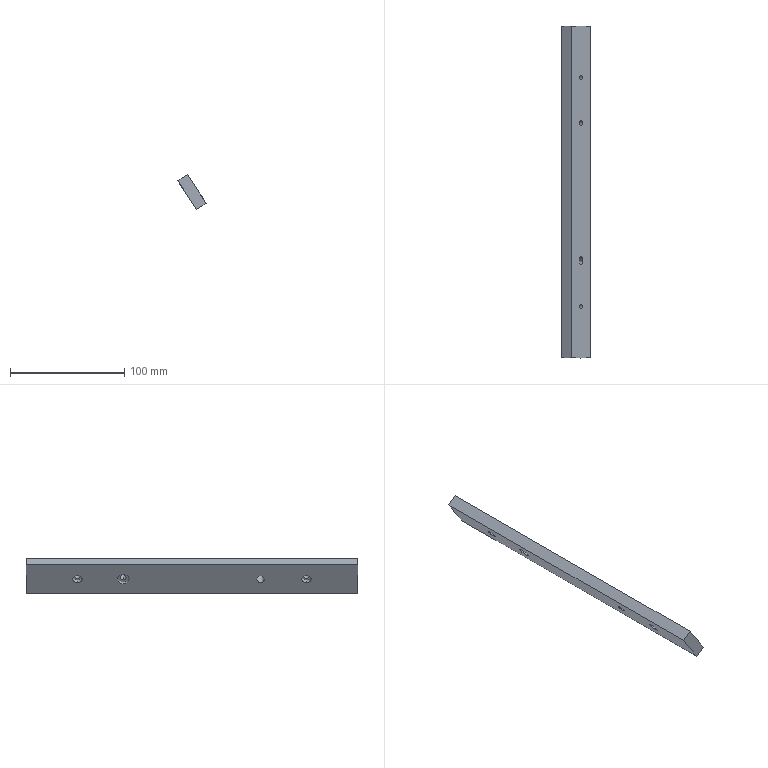Component | SolidWorks | NewSuctionCupGroup-1_SuctionCupMountingPlate-1 | 1 solid | 23 faces | box 24.78 x 290 x 30.58 mm | volume 85630 mm3 | cylinder 14 | plane 9 | commonest cylinder face diameters 8 x4 4.5 x4 5 x2 10 x2 6.8 x2
build123d program:
from build123d import *

# Parameters (mm, degrees)
SKETCH1_W                                            = 290
SKETCH1_H                                            = 30
BOSS_EXTRUDE1_DEPTH                                  = 10
M8_TAPPED_HOLE1_D                                    = 6.8
M8_TAPPED_HOLE1_DEPTH                                = 19.75
M8_TAPPED_HOLE1_TIP                                  = 2.043
SKETCH5_R                                            = 5
CUT_EXTRUDE1_DEPTH                                   = 3
SKETCH6_R                                            = 2.5
CUT_EXTRUDE2_DEPTH                                   = 146.942
HOLE_SIZE_ACCORDING_TO_THE_TYPE_OF_HEXAG_D           = 4.5
HOLE_SIZE_ACCORDING_TO_THE_TYPE_OF_HEXAG_CBORE_D     = 8
HOLE_SIZE_ACCORDING_TO_THE_TYPE_OF_HEXAG_CBORE_DEPTH = 4.6


with BuildPart() as part:
    # Sketch1 → Boss-Extrude1 (new body)
    with BuildSketch(Plane(origin=(0, 0, 0), x_dir=(1, 0, 0), z_dir=(0, 1, 0))):
        Rectangle(SKETCH1_W, SKETCH1_H)
    extrude(amount=BOSS_EXTRUDE1_DEPTH)

    # M8 Tapped Hole1
    with Locations(Plane(origin=(0, 10, 0), x_dir=(1, 0, 0), z_dir=(0, 1, 0))):
        with Locations((60, 0)):
            Hole(M8_TAPPED_HOLE1_D / 2, depth=M8_TAPPED_HOLE1_DEPTH)
            with Locations((0, 0, -(M8_TAPPED_HOLE1_DEPTH + M8_TAPPED_HOLE1_TIP / 2))):  # 118° drill point
                Cone(0, M8_TAPPED_HOLE1_D / 2, M8_TAPPED_HOLE1_TIP, mode=Mode.SUBTRACT)

    # Sketch5 → Cut-Extrude1 (cut)
    with BuildSketch(Plane.XZ):
        with Locations(Location((-60, 0, 0), (0, 0, 270))):
            Circle(SKETCH5_R)
    extrude(amount=-CUT_EXTRUDE1_DEPTH, mode=Mode.SUBTRACT)

    # Sketch6 → Cut-Extrude2 (cut, through all)
    with BuildSketch(Plane.XZ.offset(-3)):
        with Locations(Location((-60, 0, 0), (0, 0, 270))):
            Circle(SKETCH6_R)
    extrude(amount=-CUT_EXTRUDE2_DEPTH, mode=Mode.SUBTRACT)

    # Hole Size according to the type of hexag (through all)
    with Locations(Plane(origin=(0, 0, 0), x_dir=(-1, 0, 0), z_dir=(0, -1, 0))):
        with Locations((100, 0), (-100, 0)):
            CounterBoreHole(HOLE_SIZE_ACCORDING_TO_THE_TYPE_OF_HEXAG_D / 2, HOLE_SIZE_ACCORDING_TO_THE_TYPE_OF_HEXAG_CBORE_D / 2, HOLE_SIZE_ACCORDING_TO_THE_TYPE_OF_HEXAG_CBORE_DEPTH)


solid = part.part

# Placed as in the assembly
solid = solid.moved(Location((-81.422, -40.454, -24.035), (0, -33.165, -90)))
STEP:
#1=COLOUR_RGB('',0.7922,0.8196,0.9333);
#2=FILL_AREA_STYLE_COLOUR('',#1);
#3=FILL_AREA_STYLE('',(#2));
#4=SURFACE_STYLE_FILL_AREA(#3);
#5=SURFACE_SIDE_STYLE('',(#4));
#6=SURFACE_STYLE_USAGE(.BOTH.,#5);
#7=PRESENTATION_STYLE_ASSIGNMENT((#6));
#8=CARTESIAN_POINT('',(-3.14,2.344,-0.7154));
#9=VERTEX_POINT('',#8);
#10=CARTESIAN_POINT('',(-2.968,2.344,-0.979));
#11=VERTEX_POINT('',#10);
#12=CARTESIAN_POINT('',(-3.054,2.344,-0.8472));
#13=DIRECTION('',(-0.8371,0.,-0.5471));
#14=DIRECTION('',(0.5471,-0.,-0.8371));
#15=AXIS2_PLACEMENT_3D('',#12,#13,#14);
#16=CIRCLE('',#15,0.1575);
#17=EDGE_CURVE('',#9,#11,#16,.T.);
#18=ORIENTED_EDGE('',*,*,#17,.F.);
#19=CARTESIAN_POINT('',(-3.292,2.344,-0.8144));
#20=VERTEX_POINT('',#19);
#21=CARTESIAN_POINT('',(-3.292,2.344,-0.8144));
#22=DIRECTION('',(-0.8371,0.,-0.5471));
#23=VECTOR('',#22,39.37);
#24=LINE('',#21,#23);
#25=EDGE_CURVE('',#9,#20,#24,.T.);
#26=ORIENTED_EDGE('',*,*,#25,.T.);
#27=CARTESIAN_POINT('',(-3.119,2.344,-1.078));
#28=VERTEX_POINT('',#27);
#29=CARTESIAN_POINT('',(-3.206,2.344,-0.9462));
#30=DIRECTION('',(-0.8371,0.,-0.5471));
#31=DIRECTION('',(0.5471,-0.,-0.8371));
#32=AXIS2_PLACEMENT_3D('',#29,#30,#31);
#33=CIRCLE('',#32,0.1575);
#34=EDGE_CURVE('',#20,#28,#33,.T.);
#35=ORIENTED_EDGE('',*,*,#34,.T.);
#36=CARTESIAN_POINT('',(-3.119,2.344,-1.078));
#37=DIRECTION('',(-0.8371,0.,-0.5471));
#38=VECTOR('',#37,39.37);
#39=LINE('',#36,#38);
#40=EDGE_CURVE('',#11,#28,#39,.T.);
#41=ORIENTED_EDGE('',*,*,#40,.F.);
#42=EDGE_LOOP('',(#18,#26,#35,#41));
#43=FACE_OUTER_BOUND('',#42,.T.);
#44=CARTESIAN_POINT('',(-3.206,2.344,-0.9462));
#45=DIRECTION('',(-0.8371,0.,-0.5471));
#46=DIRECTION('',(0.5471,-0.,-0.8371));
#47=AXIS2_PLACEMENT_3D('',#44,#45,#46);
#48=CYLINDRICAL_SURFACE('',#47,0.1575);
#49=ADVANCED_FACE('',(#43),#48,.F.);
#50=CARTESIAN_POINT('',(-2.924,2.344,-0.6567));
#51=VERTEX_POINT('',#50);
#52=CARTESIAN_POINT('',(-2.828,2.344,-0.805));
#53=VERTEX_POINT('',#52);
#54=CARTESIAN_POINT('',(-2.876,2.344,-0.7309));
#55=DIRECTION('',(-0.8371,0.,-0.5471));
#56=DIRECTION('',(0.5471,-0.,-0.8371));
#57=AXIS2_PLACEMENT_3D('',#54,#55,#56);
#58=CIRCLE('',#57,0.08858);
#59=EDGE_CURVE('',#51,#53,#58,.T.);
#60=ORIENTED_EDGE('',*,*,#59,.F.);
#61=CARTESIAN_POINT('',(-3.102,2.344,-0.773));
#62=VERTEX_POINT('',#61);
#63=CARTESIAN_POINT('',(-3.254,2.344,-0.8721));
#64=DIRECTION('',(-0.8371,0.,-0.5471));
#65=VECTOR('',#64,39.37);
#66=LINE('',#63,#65);
#67=EDGE_CURVE('',#51,#62,#66,.T.);
#68=ORIENTED_EDGE('',*,*,#67,.T.);
#69=CARTESIAN_POINT('',(-3.006,2.344,-0.9213));
#70=VERTEX_POINT('',#69);
#71=CARTESIAN_POINT('',(-3.054,2.344,-0.8472));
#72=DIRECTION('',(-0.8371,0.,-0.5471));
#73=DIRECTION('',(0.5471,-0.,-0.8371));
#74=AXIS2_PLACEMENT_3D('',#71,#72,#73);
#75=CIRCLE('',#74,0.08858);
#76=EDGE_CURVE('',#62,#70,#75,.T.);
#77=ORIENTED_EDGE('',*,*,#76,.T.);
#78=CARTESIAN_POINT('',(-3.157,2.344,-1.02));
#79=DIRECTION('',(-0.8371,0.,-0.5471));
#80=VECTOR('',#79,39.37);
#81=LINE('',#78,#80);
#82=EDGE_CURVE('',#53,#70,#81,.T.);
#83=ORIENTED_EDGE('',*,*,#82,.F.);
#84=EDGE_LOOP('',(#60,#68,#77,#83));
#85=FACE_OUTER_BOUND('',#84,.T.);
#86=CARTESIAN_POINT('',(-3.206,2.344,-0.9462));
#87=DIRECTION('',(-0.8371,0.,-0.5471));
#88=DIRECTION('',(0.5471,-0.,-0.8371));
#89=AXIS2_PLACEMENT_3D('',#86,#87,#88);
#90=CYLINDRICAL_SURFACE('',#89,0.08858);
#91=ADVANCED_FACE('',(#85),#90,.F.);
#92=CARTESIAN_POINT('',(-3.14,-5.53,-0.7154));
#93=VERTEX_POINT('',#92);
#94=CARTESIAN_POINT('',(-2.968,-5.53,-0.979));
#95=VERTEX_POINT('',#94);
#96=CARTESIAN_POINT('',(-3.054,-5.53,-0.8472));
#97=DIRECTION('',(-0.8371,0.,-0.5471));
#98=DIRECTION('',(0.5471,0.,-0.8371));
#99=AXIS2_PLACEMENT_3D('',#96,#97,#98);
#100=CIRCLE('',#99,0.1575);
#101=EDGE_CURVE('',#93,#95,#100,.T.);
#102=ORIENTED_EDGE('',*,*,#101,.F.);
#103=CARTESIAN_POINT('',(-3.292,-5.53,-0.8144));
#104=VERTEX_POINT('',#103);
#105=CARTESIAN_POINT('',(-3.292,-5.53,-0.8144));
#106=DIRECTION('',(-0.8371,0.,-0.5471));
#107=VECTOR('',#106,39.37);
#108=LINE('',#105,#107);
#109=EDGE_CURVE('',#93,#104,#108,.T.);
#110=ORIENTED_EDGE('',*,*,#109,.T.);
#111=CARTESIAN_POINT('',(-3.119,-5.53,-1.078));
#112=VERTEX_POINT('',#111);
#113=CARTESIAN_POINT('',(-3.206,-5.53,-0.9462));
#114=DIRECTION('',(-0.8371,0.,-0.5471));
#115=DIRECTION('',(0.5471,0.,-0.8371));
#116=AXIS2_PLACEMENT_3D('',#113,#114,#115);
#117=CIRCLE('',#116,0.1575);
#118=EDGE_CURVE('',#104,#112,#117,.T.);
#119=ORIENTED_EDGE('',*,*,#118,.T.);
#120=CARTESIAN_POINT('',(-3.119,-5.53,-1.078));
#121=DIRECTION('',(-0.8371,0.,-0.5471));
#122=VECTOR('',#121,39.37);
#123=LINE('',#120,#122);
#124=EDGE_CURVE('',#95,#112,#123,.T.);
#125=ORIENTED_EDGE('',*,*,#124,.F.);
#126=EDGE_LOOP('',(#102,#110,#119,#125));
#127=FACE_OUTER_BOUND('',#126,.T.);
#128=CARTESIAN_POINT('',(-3.206,-5.53,-0.9462));
#129=DIRECTION('',(-0.8371,0.,-0.5471));
#130=DIRECTION('',(0.5471,0.,-0.8371));
#131=AXIS2_PLACEMENT_3D('',#128,#129,#130);
#132=CYLINDRICAL_SURFACE('',#131,0.1575);
#133=ADVANCED_FACE('',(#127),#132,.F.);
#134=CARTESIAN_POINT('',(-2.924,-5.53,-0.6567));
#135=VERTEX_POINT('',#134);
#136=CARTESIAN_POINT('',(-2.828,-5.53,-0.805));
#137=VERTEX_POINT('',#136);
#138=CARTESIAN_POINT('',(-2.876,-5.53,-0.7309));
#139=DIRECTION('',(-0.8371,0.,-0.5471));
#140=DIRECTION('',(0.5471,0.,-0.8371));
#141=AXIS2_PLACEMENT_3D('',#138,#139,#140);
#142=CIRCLE('',#141,0.08858);
#143=EDGE_CURVE('',#135,#137,#142,.T.);
#144=ORIENTED_EDGE('',*,*,#143,.F.);
#145=CARTESIAN_POINT('',(-3.102,-5.53,-0.773));
#146=VERTEX_POINT('',#145);
#147=CARTESIAN_POINT('',(-3.254,-5.53,-0.8721));
#148=DIRECTION('',(-0.8371,0.,-0.5471));
#149=VECTOR('',#148,39.37);
#150=LINE('',#147,#149);
#151=EDGE_CURVE('',#135,#146,#150,.T.);
#152=ORIENTED_EDGE('',*,*,#151,.T.);
#153=CARTESIAN_POINT('',(-3.006,-5.53,-0.9213));
#154=VERTEX_POINT('',#153);
#155=CARTESIAN_POINT('',(-3.054,-5.53,-0.8472));
#156=DIRECTION('',(-0.8371,0.,-0.5471));
#157=DIRECTION('',(0.5471,0.,-0.8371));
#158=AXIS2_PLACEMENT_3D('',#155,#156,#157);
#159=CIRCLE('',#158,0.08858);
#160=EDGE_CURVE('',#146,#154,#159,.T.);
#161=ORIENTED_EDGE('',*,*,#160,.T.);
#162=CARTESIAN_POINT('',(-3.157,-5.53,-1.02));
#163=DIRECTION('',(-0.8371,0.,-0.5471));
#164=VECTOR('',#163,39.37);
#165=LINE('',#162,#164);
#166=EDGE_CURVE('',#137,#154,#165,.T.);
#167=ORIENTED_EDGE('',*,*,#166,.F.);
#168=EDGE_LOOP('',(#144,#152,#161,#167));
#169=FACE_OUTER_BOUND('',#168,.T.);
#170=CARTESIAN_POINT('',(-3.206,-5.53,-0.9462));
#171=DIRECTION('',(-0.8371,0.,-0.5471));
#172=DIRECTION('',(0.5471,0.,-0.8371));
#173=AXIS2_PLACEMENT_3D('',#170,#171,#172);
#174=CYLINDRICAL_SURFACE('',#173,0.08858);
#175=ADVANCED_FACE('',(#169),#174,.F.);
#176=CARTESIAN_POINT('',(-2.93,0.7695,-0.6485));
#177=VERTEX_POINT('',#176);
#178=CARTESIAN_POINT('',(-2.822,0.7695,-0.8133));
#179=VERTEX_POINT('',#178);
#180=CARTESIAN_POINT('',(-2.876,0.7695,-0.7309));
#181=DIRECTION('',(-0.8371,0.,-0.5471));
#182=DIRECTION('',(0.5471,-0.,-0.8371));
#183=AXIS2_PLACEMENT_3D('',#180,#181,#182);
#184=CIRCLE('',#183,0.09843);
#185=EDGE_CURVE('',#177,#179,#184,.T.);
#186=ORIENTED_EDGE('',*,*,#185,.F.);
#187=CARTESIAN_POINT('',(-3.161,0.7695,-0.7992));
#188=VERTEX_POINT('',#187);
#189=CARTESIAN_POINT('',(-2.93,0.7695,-0.6485));
#190=DIRECTION('',(-0.8371,0.,-0.5471));
#191=VECTOR('',#190,39.37);
#192=LINE('',#189,#191);
#193=EDGE_CURVE('',#177,#188,#192,.T.);
#194=ORIENTED_EDGE('',*,*,#193,.T.);
#195=CARTESIAN_POINT('',(-3.053,0.7695,-0.964));
#196=VERTEX_POINT('',#195);
#197=CARTESIAN_POINT('',(-3.107,0.7695,-0.8816));
#198=DIRECTION('',(-0.8371,0.,-0.5471));
#199=DIRECTION('',(0.5471,-0.,-0.8371));
#200=AXIS2_PLACEMENT_3D('',#197,#198,#199);
#201=CIRCLE('',#200,0.09843);
#202=EDGE_CURVE('',#188,#196,#201,.T.);
#203=ORIENTED_EDGE('',*,*,#202,.T.);
#204=CARTESIAN_POINT('',(-2.822,0.7695,-0.8133));
#205=DIRECTION('',(-0.8371,0.,-0.5471));
#206=VECTOR('',#205,39.37);
#207=LINE('',#204,#206);
#208=EDGE_CURVE('',#179,#196,#207,.T.);
#209=ORIENTED_EDGE('',*,*,#208,.F.);
#210=EDGE_LOOP('',(#186,#194,#203,#209));
#211=FACE_OUTER_BOUND('',#210,.T.);
#212=CARTESIAN_POINT('',(-2.876,0.7695,-0.7309));
#213=DIRECTION('',(-0.8371,0.,-0.5471));
#214=DIRECTION('',(0.5471,-0.,-0.8371));
#215=AXIS2_PLACEMENT_3D('',#212,#213,#214);
#216=CYLINDRICAL_SURFACE('',#215,0.09843);
#217=ADVANCED_FACE('',(#211),#216,.F.);
#218=CARTESIAN_POINT('',(-3.214,0.7695,-0.7169));
#219=VERTEX_POINT('',#218);
#220=CARTESIAN_POINT('',(-2.999,0.7695,-1.046));
#221=VERTEX_POINT('',#220);
#222=CARTESIAN_POINT('',(-3.107,0.7695,-0.8816));
#223=DIRECTION('',(-0.8371,0.,-0.5471));
#224=DIRECTION('',(0.5471,-0.,-0.8371));
#225=AXIS2_PLACEMENT_3D('',#222,#223,#224);
#226=CIRCLE('',#225,0.1969);
#227=EDGE_CURVE('',#219,#221,#226,.T.);
#228=ORIENTED_EDGE('',*,*,#227,.F.);
#229=CARTESIAN_POINT('',(-3.313,0.7695,-0.7815));
#230=VERTEX_POINT('',#229);
#231=CARTESIAN_POINT('',(-3.214,0.7695,-0.7169));
#232=DIRECTION('',(-0.8371,0.,-0.5471));
#233=VECTOR('',#232,39.37);
#234=LINE('',#231,#233);
#235=EDGE_CURVE('',#219,#230,#234,.T.);
#236=ORIENTED_EDGE('',*,*,#235,.T.);
#237=CARTESIAN_POINT('',(-3.098,0.7695,-1.111));
#238=VERTEX_POINT('',#237);
#239=CARTESIAN_POINT('',(-3.206,0.7695,-0.9462));
#240=DIRECTION('',(-0.8371,0.,-0.5471));
#241=DIRECTION('',(0.5471,-0.,-0.8371));
#242=AXIS2_PLACEMENT_3D('',#239,#240,#241);
#243=CIRCLE('',#242,0.1969);
#244=EDGE_CURVE('',#230,#238,#243,.T.);
#245=ORIENTED_EDGE('',*,*,#244,.T.);
#246=CARTESIAN_POINT('',(-2.999,0.7695,-1.046));
#247=DIRECTION('',(-0.8371,0.,-0.5471));
#248=VECTOR('',#247,39.37);
#249=LINE('',#246,#248);
#250=EDGE_CURVE('',#221,#238,#249,.T.);
#251=ORIENTED_EDGE('',*,*,#250,.F.);
#252=EDGE_LOOP('',(#228,#236,#245,#251));
#253=FACE_OUTER_BOUND('',#252,.T.);
#254=CARTESIAN_POINT('',(-3.107,0.7695,-0.8816));
#255=DIRECTION('',(-0.8371,0.,-0.5471));
#256=DIRECTION('',(0.5471,-0.,-0.8371));
#257=AXIS2_PLACEMENT_3D('',#254,#255,#256);
#258=CYLINDRICAL_SURFACE('',#257,0.1969);
#259=ADVANCED_FACE('',(#253),#258,.F.);
#260=CARTESIAN_POINT('',(-3.279,-3.955,-0.8342));
#261=VERTEX_POINT('',#260);
#262=CARTESIAN_POINT('',(-3.132,-3.955,-1.058));
#263=VERTEX_POINT('',#262);
#264=CARTESIAN_POINT('',(-3.206,-3.955,-0.9462));
#265=DIRECTION('',(-0.8371,0.,-0.5471));
#266=DIRECTION('',(0.5471,0.,-0.8371));
#267=AXIS2_PLACEMENT_3D('',#264,#265,#266);
#268=CIRCLE('',#267,0.1339);
#269=EDGE_CURVE('',#261,#263,#268,.T.);
#270=ORIENTED_EDGE('',*,*,#269,.T.);
#271=CARTESIAN_POINT('',(-2.803,-3.955,-0.8429));
#272=VERTEX_POINT('',#271);
#273=CARTESIAN_POINT('',(-2.803,-3.955,-0.8429));
#274=DIRECTION('',(0.8371,-0.,0.5471));
#275=VECTOR('',#274,39.37);
#276=LINE('',#273,#275);
#277=EDGE_CURVE('',#263,#272,#276,.T.);
#278=ORIENTED_EDGE('',*,*,#277,.T.);
#279=CARTESIAN_POINT('',(-2.949,-3.955,-0.6188));
#280=VERTEX_POINT('',#279);
#281=CARTESIAN_POINT('',(-2.876,-3.955,-0.7309));
#282=DIRECTION('',(0.8371,-0.,0.5471));
#283=DIRECTION('',(-0.5471,0.,0.8371));
#284=AXIS2_PLACEMENT_3D('',#281,#282,#283);
#285=CIRCLE('',#284,0.1339);
#286=EDGE_CURVE('',#272,#280,#285,.T.);
#287=ORIENTED_EDGE('',*,*,#286,.T.);
#288=CARTESIAN_POINT('',(-2.949,-3.955,-0.6188));
#289=DIRECTION('',(0.8371,-0.,0.5471));
#290=VECTOR('',#289,39.37);
#291=LINE('',#288,#290);
#292=EDGE_CURVE('',#261,#280,#291,.T.);
#293=ORIENTED_EDGE('',*,*,#292,.F.);
#294=EDGE_LOOP('',(#270,#278,#287,#293));
#295=FACE_OUTER_BOUND('',#294,.T.);
#296=CARTESIAN_POINT('',(-2.876,-3.955,-0.7309));
#297=DIRECTION('',(0.8371,-0.,0.5471));
#298=DIRECTION('',(-0.5471,0.,0.8371));
#299=AXIS2_PLACEMENT_3D('',#296,#297,#298);
#300=CYLINDRICAL_SURFACE('',#299,0.1339);
#301=ADVANCED_FACE('',(#295),#300,.F.);
#302=CARTESIAN_POINT('',(-3.529,-7.301,-0.4519));
#303=VERTEX_POINT('',#302);
#304=CARTESIAN_POINT('',(-2.883,-7.301,-1.441));
#305=VERTEX_POINT('',#304);
#306=CARTESIAN_POINT('',(-3.529,-7.301,-0.4519));
#307=DIRECTION('',(0.5471,-0.,-0.8371));
#308=VECTOR('',#307,39.37);
#309=LINE('',#306,#308);
#310=EDGE_CURVE('',#303,#305,#309,.T.);
#311=ORIENTED_EDGE('',*,*,#310,.T.);
#312=CARTESIAN_POINT('',(-2.553,-7.301,-1.225));
#313=VERTEX_POINT('',#312);
#314=CARTESIAN_POINT('',(-2.553,-7.301,-1.225));
#315=DIRECTION('',(-0.8371,0.,-0.5471));
#316=VECTOR('',#315,39.37);
#317=LINE('',#314,#316);
#318=EDGE_CURVE('',#313,#305,#317,.T.);
#319=ORIENTED_EDGE('',*,*,#318,.F.);
#320=CARTESIAN_POINT('',(-3.199,-7.301,-0.2365));
#321=VERTEX_POINT('',#320);
#322=CARTESIAN_POINT('',(-3.199,-7.301,-0.2365));
#323=DIRECTION('',(0.5471,-0.,-0.8371));
#324=VECTOR('',#323,39.37);
#325=LINE('',#322,#324);
#326=EDGE_CURVE('',#321,#313,#325,.T.);
#327=ORIENTED_EDGE('',*,*,#326,.F.);
#328=CARTESIAN_POINT('',(-3.199,-7.301,-0.2365));
#329=DIRECTION('',(-0.8371,0.,-0.5471));
#330=VECTOR('',#329,39.37);
#331=LINE('',#328,#330);
#332=EDGE_CURVE('',#321,#303,#331,.T.);
#333=ORIENTED_EDGE('',*,*,#332,.T.);
#334=EDGE_LOOP('',(#311,#319,#327,#333));
#335=FACE_OUTER_BOUND('',#334,.T.);
#336=CARTESIAN_POINT('',(-3.199,-7.301,-0.2365));
#337=DIRECTION('',(0.,1.,-0.));
#338=DIRECTION('',(-0.5471,0.,0.8371));
#339=AXIS2_PLACEMENT_3D('',#336,#337,#338);
#340=PLANE('',#339);
#341=ADVANCED_FACE('',(#335),#340,.F.);
#342=CARTESIAN_POINT('',(-2.883,4.116,-1.441));
#343=VERTEX_POINT('',#342);
#344=CARTESIAN_POINT('',(-2.883,4.116,-1.441));
#345=DIRECTION('',(0.,1.,-0.));
#346=VECTOR('',#345,39.37);
#347=LINE('',#344,#346);
#348=EDGE_CURVE('',#305,#343,#347,.T.);
#349=ORIENTED_EDGE('',*,*,#348,.T.);
#350=CARTESIAN_POINT('',(-2.553,4.116,-1.225));
#351=VERTEX_POINT('',#350);
#352=CARTESIAN_POINT('',(-2.553,4.116,-1.225));
#353=DIRECTION('',(-0.8371,0.,-0.5471));
#354=VECTOR('',#353,39.37);
#355=LINE('',#352,#354);
#356=EDGE_CURVE('',#351,#343,#355,.T.);
#357=ORIENTED_EDGE('',*,*,#356,.F.);
#358=CARTESIAN_POINT('',(-2.553,4.116,-1.225));
#359=DIRECTION('',(0.,1.,-0.));
#360=VECTOR('',#359,39.37);
#361=LINE('',#358,#360);
#362=EDGE_CURVE('',#313,#351,#361,.T.);
#363=ORIENTED_EDGE('',*,*,#362,.F.);
#364=ORIENTED_EDGE('',*,*,#318,.T.);
#365=EDGE_LOOP('',(#349,#357,#363,#364));
#366=FACE_OUTER_BOUND('',#365,.T.);
#367=CARTESIAN_POINT('',(-2.553,4.116,-1.225));
#368=DIRECTION('',(-0.5471,0.,0.8371));
#369=DIRECTION('',(-0.,-1.,0.));
#370=AXIS2_PLACEMENT_3D('',#367,#368,#369);
#371=PLANE('',#370);
#372=ADVANCED_FACE('',(#366),#371,.F.);
#373=CARTESIAN_POINT('',(-3.529,4.116,-0.4519));
#374=VERTEX_POINT('',#373);
#375=CARTESIAN_POINT('',(-3.529,4.116,-0.4519));
#376=DIRECTION('',(-0.5471,0.,0.8371));
#377=VECTOR('',#376,39.37);
#378=LINE('',#375,#377);
#379=EDGE_CURVE('',#343,#374,#378,.T.);
#380=ORIENTED_EDGE('',*,*,#379,.T.);
#381=CARTESIAN_POINT('',(-3.199,4.116,-0.2365));
#382=VERTEX_POINT('',#381);
#383=CARTESIAN_POINT('',(-3.199,4.116,-0.2365));
#384=DIRECTION('',(-0.8371,0.,-0.5471));
#385=VECTOR('',#384,39.37);
#386=LINE('',#383,#385);
#387=EDGE_CURVE('',#382,#374,#386,.T.);
#388=ORIENTED_EDGE('',*,*,#387,.F.);
#389=CARTESIAN_POINT('',(-3.199,4.116,-0.2365));
#390=DIRECTION('',(-0.5471,0.,0.8371));
#391=VECTOR('',#390,39.37);
#392=LINE('',#389,#391);
#393=EDGE_CURVE('',#351,#382,#392,.T.);
#394=ORIENTED_EDGE('',*,*,#393,.F.);
#395=ORIENTED_EDGE('',*,*,#356,.T.);
#396=EDGE_LOOP('',(#380,#388,#394,#395));
#397=FACE_OUTER_BOUND('',#396,.T.);
#398=CARTESIAN_POINT('',(-3.199,4.116,-0.2365));
#399=DIRECTION('',(-0.,-1.,0.));
#400=DIRECTION('',(0.5471,-0.,-0.8371));
#401=AXIS2_PLACEMENT_3D('',#398,#399,#400);
#402=PLANE('',#401);
#403=ADVANCED_FACE('',(#397),#402,.F.);
#404=CARTESIAN_POINT('',(-3.529,4.116,-0.4519));
#405=DIRECTION('',(-0.,-1.,0.));
#406=VECTOR('',#405,39.37);
#407=LINE('',#404,#406);
#408=EDGE_CURVE('',#374,#303,#407,.T.);
#409=ORIENTED_EDGE('',*,*,#408,.T.);
#410=ORIENTED_EDGE('',*,*,#332,.F.);
#411=CARTESIAN_POINT('',(-3.199,4.116,-0.2365));
#412=DIRECTION('',(-0.,-1.,0.));
#413=VECTOR('',#412,39.37);
#414=LINE('',#411,#413);
#415=EDGE_CURVE('',#382,#321,#414,.T.);
#416=ORIENTED_EDGE('',*,*,#415,.F.);
#417=ORIENTED_EDGE('',*,*,#387,.T.);
#418=EDGE_LOOP('',(#409,#410,#416,#417));
#419=FACE_OUTER_BOUND('',#418,.T.);
#420=CARTESIAN_POINT('',(-3.199,4.116,-0.2365));
#421=DIRECTION('',(0.5471,-0.,-0.8371));
#422=DIRECTION('',(0.,1.,-0.));
#423=AXIS2_PLACEMENT_3D('',#420,#421,#422);
#424=PLANE('',#423);
#425=ADVANCED_FACE('',(#419),#424,.F.);
#426=CARTESIAN_POINT('',(-2.876,2.344,-0.7309));
#427=DIRECTION('',(-0.8371,0.,-0.5471));
#428=DIRECTION('',(0.5471,-0.,-0.8371));
#429=AXIS2_PLACEMENT_3D('',#426,#427,#428);
#430=CIRCLE('',#429,0.08858);
#431=EDGE_CURVE('',#53,#51,#430,.T.);
#432=ORIENTED_EDGE('',*,*,#431,.T.);
#433=ORIENTED_EDGE('',*,*,#59,.T.);
#434=EDGE_LOOP('',(#432,#433));
#435=FACE_BOUND('',#434,.T.);
#436=CARTESIAN_POINT('',(-2.876,-5.53,-0.7309));
#437=DIRECTION('',(-0.8371,0.,-0.5471));
#438=DIRECTION('',(0.5471,0.,-0.8371));
#439=AXIS2_PLACEMENT_3D('',#436,#437,#438);
#440=CIRCLE('',#439,0.08858);
#441=EDGE_CURVE('',#137,#135,#440,.T.);
#442=ORIENTED_EDGE('',*,*,#441,.T.);
#443=ORIENTED_EDGE('',*,*,#143,.T.);
#444=EDGE_LOOP('',(#442,#443));
#445=FACE_BOUND('',#444,.T.);
#446=CARTESIAN_POINT('',(-2.876,0.7695,-0.7309));
#447=DIRECTION('',(-0.8371,0.,-0.5471));
#448=DIRECTION('',(0.5471,-0.,-0.8371));
#449=AXIS2_PLACEMENT_3D('',#446,#447,#448);
#450=CIRCLE('',#449,0.09843);
#451=EDGE_CURVE('',#179,#177,#450,.T.);
#452=ORIENTED_EDGE('',*,*,#451,.T.);
#453=ORIENTED_EDGE('',*,*,#185,.T.);
#454=EDGE_LOOP('',(#452,#453));
#455=FACE_BOUND('',#454,.T.);
#456=CARTESIAN_POINT('',(-2.876,-3.955,-0.7309));
#457=DIRECTION('',(0.8371,-0.,0.5471));
#458=DIRECTION('',(-0.5471,0.,0.8371));
#459=AXIS2_PLACEMENT_3D('',#456,#457,#458);
#460=CIRCLE('',#459,0.1339);
#461=EDGE_CURVE('',#280,#272,#460,.T.);
#462=ORIENTED_EDGE('',*,*,#461,.F.);
#463=ORIENTED_EDGE('',*,*,#286,.F.);
#464=EDGE_LOOP('',(#462,#463));
#465=FACE_BOUND('',#464,.T.);
#466=ORIENTED_EDGE('',*,*,#326,.T.);
#467=ORIENTED_EDGE('',*,*,#362,.T.);
#468=ORIENTED_EDGE('',*,*,#393,.T.);
#469=ORIENTED_EDGE('',*,*,#415,.T.);
#470=EDGE_LOOP('',(#466,#467,#468,#469));
#471=FACE_OUTER_BOUND('',#470,.T.);
#472=CARTESIAN_POINT('',(-2.876,-1.593,-0.7309));
#473=DIRECTION('',(-0.8371,0.,-0.5471));
#474=DIRECTION('',(0.5471,-0.,-0.8371));
#475=AXIS2_PLACEMENT_3D('',#472,#473,#474);
#476=PLANE('',#475);
#477=ADVANCED_FACE('',(#435,#445,#455,#465,#471),#476,.F.);
#478=CARTESIAN_POINT('',(-3.206,2.344,-0.9462));
#479=DIRECTION('',(-0.8371,0.,-0.5471));
#480=DIRECTION('',(0.5471,-0.,-0.8371));
#481=AXIS2_PLACEMENT_3D('',#478,#479,#480);
#482=CIRCLE('',#481,0.1575);
#483=EDGE_CURVE('',#28,#20,#482,.T.);
#484=ORIENTED_EDGE('',*,*,#483,.F.);
#485=ORIENTED_EDGE('',*,*,#34,.F.);
#486=EDGE_LOOP('',(#484,#485));
#487=FACE_BOUND('',#486,.T.);
#488=CARTESIAN_POINT('',(-3.206,-5.53,-0.9462));
#489=DIRECTION('',(-0.8371,0.,-0.5471));
#490=DIRECTION('',(0.5471,0.,-0.8371));
#491=AXIS2_PLACEMENT_3D('',#488,#489,#490);
#492=CIRCLE('',#491,0.1575);
#493=EDGE_CURVE('',#112,#104,#492,.T.);
#494=ORIENTED_EDGE('',*,*,#493,.F.);
#495=ORIENTED_EDGE('',*,*,#118,.F.);
#496=EDGE_LOOP('',(#494,#495));
#497=FACE_BOUND('',#496,.T.);
#498=CARTESIAN_POINT('',(-3.206,0.7695,-0.9462));
#499=DIRECTION('',(-0.8371,0.,-0.5471));
#500=DIRECTION('',(0.5471,-0.,-0.8371));
#501=AXIS2_PLACEMENT_3D('',#498,#499,#500);
#502=CIRCLE('',#501,0.1969);
#503=EDGE_CURVE('',#238,#230,#502,.T.);
#504=ORIENTED_EDGE('',*,*,#503,.F.);
#505=ORIENTED_EDGE('',*,*,#244,.F.);
#506=EDGE_LOOP('',(#504,#505));
#507=FACE_BOUND('',#506,.T.);
#508=ORIENTED_EDGE('',*,*,#269,.F.);
#509=CARTESIAN_POINT('',(-3.206,-3.955,-0.9462));
#510=DIRECTION('',(-0.8371,0.,-0.5471));
#511=DIRECTION('',(0.5471,0.,-0.8371));
#512=AXIS2_PLACEMENT_3D('',#509,#510,#511);
#513=CIRCLE('',#512,0.1339);
#514=EDGE_CURVE('',#263,#261,#513,.T.);
#515=ORIENTED_EDGE('',*,*,#514,.F.);
#516=EDGE_LOOP('',(#508,#515));
#517=FACE_BOUND('',#516,.T.);
#518=ORIENTED_EDGE('',*,*,#310,.F.);
#519=ORIENTED_EDGE('',*,*,#408,.F.);
#520=ORIENTED_EDGE('',*,*,#379,.F.);
#521=ORIENTED_EDGE('',*,*,#348,.F.);
#522=EDGE_LOOP('',(#518,#519,#520,#521));
#523=FACE_OUTER_BOUND('',#522,.T.);
#524=CARTESIAN_POINT('',(-3.206,-1.593,-0.9462));
#525=DIRECTION('',(-0.8371,0.,-0.5471));
#526=DIRECTION('',(0.5471,-0.,-0.8371));
#527=AXIS2_PLACEMENT_3D('',#524,#525,#526);
#528=PLANE('',#527);
#529=ADVANCED_FACE('',(#487,#497,#507,#517,#523),#528,.T.);
#530=ORIENTED_EDGE('',*,*,#277,.F.);
#531=ORIENTED_EDGE('',*,*,#514,.T.);
#532=ORIENTED_EDGE('',*,*,#292,.T.);
#533=ORIENTED_EDGE('',*,*,#461,.T.);
#534=EDGE_LOOP('',(#530,#531,#532,#533));
#535=FACE_OUTER_BOUND('',#534,.T.);
#536=CARTESIAN_POINT('',(-2.876,-3.955,-0.7309));
#537=DIRECTION('',(0.8371,-0.,0.5471));
#538=DIRECTION('',(-0.5471,0.,0.8371));
#539=AXIS2_PLACEMENT_3D('',#536,#537,#538);
#540=CYLINDRICAL_SURFACE('',#539,0.1339);
#541=ADVANCED_FACE('',(#535),#540,.F.);
#542=ORIENTED_EDGE('',*,*,#235,.F.);
#543=CARTESIAN_POINT('',(-3.107,0.7695,-0.8816));
#544=DIRECTION('',(-0.8371,0.,-0.5471));
#545=DIRECTION('',(0.5471,-0.,-0.8371));
#546=AXIS2_PLACEMENT_3D('',#543,#544,#545);
#547=CIRCLE('',#546,0.1969);
#548=EDGE_CURVE('',#221,#219,#547,.T.);
#549=ORIENTED_EDGE('',*,*,#548,.F.);
#550=ORIENTED_EDGE('',*,*,#250,.T.);
#551=ORIENTED_EDGE('',*,*,#503,.T.);
#552=EDGE_LOOP('',(#542,#549,#550,#551));
#553=FACE_OUTER_BOUND('',#552,.T.);
#554=CARTESIAN_POINT('',(-3.107,0.7695,-0.8816));
#555=DIRECTION('',(-0.8371,0.,-0.5471));
#556=DIRECTION('',(0.5471,-0.,-0.8371));
#557=AXIS2_PLACEMENT_3D('',#554,#555,#556);
#558=CYLINDRICAL_SURFACE('',#557,0.1969);
#559=ADVANCED_FACE('',(#553),#558,.F.);
#560=CARTESIAN_POINT('',(-3.107,0.7695,-0.8816));
#561=DIRECTION('',(-0.8371,0.,-0.5471));
#562=DIRECTION('',(0.5471,-0.,-0.8371));
#563=AXIS2_PLACEMENT_3D('',#560,#561,#562);
#564=CIRCLE('',#563,0.09843);
#565=EDGE_CURVE('',#196,#188,#564,.T.);
#566=ORIENTED_EDGE('',*,*,#565,.F.);
#567=ORIENTED_EDGE('',*,*,#202,.F.);
#568=EDGE_LOOP('',(#566,#567));
#569=FACE_BOUND('',#568,.T.);
#570=ORIENTED_EDGE('',*,*,#548,.T.);
#571=ORIENTED_EDGE('',*,*,#227,.T.);
#572=EDGE_LOOP('',(#570,#571));
#573=FACE_OUTER_BOUND('',#572,.T.);
#574=CARTESIAN_POINT('',(-3.107,0.7695,-0.8816));
#575=DIRECTION('',(-0.8371,0.,-0.5471));
#576=DIRECTION('',(0.5471,-0.,-0.8371));
#577=AXIS2_PLACEMENT_3D('',#574,#575,#576);
#578=PLANE('',#577);
#579=ADVANCED_FACE('',(#569,#573),#578,.T.);
#580=ORIENTED_EDGE('',*,*,#193,.F.);
#581=ORIENTED_EDGE('',*,*,#451,.F.);
#582=ORIENTED_EDGE('',*,*,#208,.T.);
#583=ORIENTED_EDGE('',*,*,#565,.T.);
#584=EDGE_LOOP('',(#580,#581,#582,#583));
#585=FACE_OUTER_BOUND('',#584,.T.);
#586=CARTESIAN_POINT('',(-2.876,0.7695,-0.7309));
#587=DIRECTION('',(-0.8371,0.,-0.5471));
#588=DIRECTION('',(0.5471,-0.,-0.8371));
#589=AXIS2_PLACEMENT_3D('',#586,#587,#588);
#590=CYLINDRICAL_SURFACE('',#589,0.09843);
#591=ADVANCED_FACE('',(#585),#590,.F.);
#592=ORIENTED_EDGE('',*,*,#151,.F.);
#593=ORIENTED_EDGE('',*,*,#441,.F.);
#594=ORIENTED_EDGE('',*,*,#166,.T.);
#595=CARTESIAN_POINT('',(-3.054,-5.53,-0.8472));
#596=DIRECTION('',(-0.8371,0.,-0.5471));
#597=DIRECTION('',(0.5471,0.,-0.8371));
#598=AXIS2_PLACEMENT_3D('',#595,#596,#597);
#599=CIRCLE('',#598,0.08858);
#600=EDGE_CURVE('',#154,#146,#599,.T.);
#601=ORIENTED_EDGE('',*,*,#600,.T.);
#602=EDGE_LOOP('',(#592,#593,#594,#601));
#603=FACE_OUTER_BOUND('',#602,.T.);
#604=CARTESIAN_POINT('',(-3.206,-5.53,-0.9462));
#605=DIRECTION('',(-0.8371,0.,-0.5471));
#606=DIRECTION('',(0.5471,0.,-0.8371));
#607=AXIS2_PLACEMENT_3D('',#604,#605,#606);
#608=CYLINDRICAL_SURFACE('',#607,0.08858);
#609=ADVANCED_FACE('',(#603),#608,.F.);
#610=ORIENTED_EDGE('',*,*,#600,.F.);
#611=ORIENTED_EDGE('',*,*,#160,.F.);
#612=EDGE_LOOP('',(#610,#611));
#613=FACE_BOUND('',#612,.T.);
#614=CARTESIAN_POINT('',(-3.054,-5.53,-0.8472));
#615=DIRECTION('',(-0.8371,0.,-0.5471));
#616=DIRECTION('',(0.5471,0.,-0.8371));
#617=AXIS2_PLACEMENT_3D('',#614,#615,#616);
#618=CIRCLE('',#617,0.1575);
#619=EDGE_CURVE('',#95,#93,#618,.T.);
#620=ORIENTED_EDGE('',*,*,#619,.T.);
#621=ORIENTED_EDGE('',*,*,#101,.T.);
#622=EDGE_LOOP('',(#620,#621));
#623=FACE_OUTER_BOUND('',#622,.T.);
#624=CARTESIAN_POINT('',(-3.054,-5.618,-0.8472));
#625=DIRECTION('',(0.8371,-0.,0.5471));
#626=DIRECTION('',(-0.5471,0.,0.8371));
#627=AXIS2_PLACEMENT_3D('',#624,#625,#626);
#628=PLANE('',#627);
#629=ADVANCED_FACE('',(#613,#623),#628,.F.);
#630=ORIENTED_EDGE('',*,*,#109,.F.);
#631=ORIENTED_EDGE('',*,*,#619,.F.);
#632=ORIENTED_EDGE('',*,*,#124,.T.);
#633=ORIENTED_EDGE('',*,*,#493,.T.);
#634=EDGE_LOOP('',(#630,#631,#632,#633));
#635=FACE_OUTER_BOUND('',#634,.T.);
#636=CARTESIAN_POINT('',(-3.206,-5.53,-0.9462));
#637=DIRECTION('',(-0.8371,0.,-0.5471));
#638=DIRECTION('',(0.5471,0.,-0.8371));
#639=AXIS2_PLACEMENT_3D('',#636,#637,#638);
#640=CYLINDRICAL_SURFACE('',#639,0.1575);
#641=ADVANCED_FACE('',(#635),#640,.F.);
#642=ORIENTED_EDGE('',*,*,#67,.F.);
#643=ORIENTED_EDGE('',*,*,#431,.F.);
#644=ORIENTED_EDGE('',*,*,#82,.T.);
#645=CARTESIAN_POINT('',(-3.054,2.344,-0.8472));
#646=DIRECTION('',(-0.8371,0.,-0.5471));
#647=DIRECTION('',(0.5471,-0.,-0.8371));
#648=AXIS2_PLACEMENT_3D('',#645,#646,#647);
#649=CIRCLE('',#648,0.08858);
#650=EDGE_CURVE('',#70,#62,#649,.T.);
#651=ORIENTED_EDGE('',*,*,#650,.T.);
#652=EDGE_LOOP('',(#642,#643,#644,#651));
#653=FACE_OUTER_BOUND('',#652,.T.);
#654=CARTESIAN_POINT('',(-3.206,2.344,-0.9462));
#655=DIRECTION('',(-0.8371,0.,-0.5471));
#656=DIRECTION('',(0.5471,-0.,-0.8371));
#657=AXIS2_PLACEMENT_3D('',#654,#655,#656);
#658=CYLINDRICAL_SURFACE('',#657,0.08858);
#659=ADVANCED_FACE('',(#653),#658,.F.);
#660=ORIENTED_EDGE('',*,*,#650,.F.);
#661=ORIENTED_EDGE('',*,*,#76,.F.);
#662=EDGE_LOOP('',(#660,#661));
#663=FACE_BOUND('',#662,.T.);
#664=CARTESIAN_POINT('',(-3.054,2.344,-0.8472));
#665=DIRECTION('',(-0.8371,0.,-0.5471));
#666=DIRECTION('',(0.5471,-0.,-0.8371));
#667=AXIS2_PLACEMENT_3D('',#664,#665,#666);
#668=CIRCLE('',#667,0.1575);
#669=EDGE_CURVE('',#11,#9,#668,.T.);
#670=ORIENTED_EDGE('',*,*,#669,.T.);
#671=ORIENTED_EDGE('',*,*,#17,.T.);
#672=EDGE_LOOP('',(#670,#671));
#673=FACE_OUTER_BOUND('',#672,.T.);
#674=CARTESIAN_POINT('',(-3.054,2.256,-0.8472));
#675=DIRECTION('',(0.8371,-0.,0.5471));
#676=DIRECTION('',(-0.5471,0.,0.8371));
#677=AXIS2_PLACEMENT_3D('',#674,#675,#676);
#678=PLANE('',#677);
#679=ADVANCED_FACE('',(#663,#673),#678,.F.);
#680=ORIENTED_EDGE('',*,*,#25,.F.);
#681=ORIENTED_EDGE('',*,*,#669,.F.);
#682=ORIENTED_EDGE('',*,*,#40,.T.);
#683=ORIENTED_EDGE('',*,*,#483,.T.);
#684=EDGE_LOOP('',(#680,#681,#682,#683));
#685=FACE_OUTER_BOUND('',#684,.T.);
#686=CARTESIAN_POINT('',(-3.206,2.344,-0.9462));
#687=DIRECTION('',(-0.8371,0.,-0.5471));
#688=DIRECTION('',(0.5471,-0.,-0.8371));
#689=AXIS2_PLACEMENT_3D('',#686,#687,#688);
#690=CYLINDRICAL_SURFACE('',#689,0.1575);
#691=ADVANCED_FACE('',(#685),#690,.F.);
#692=CLOSED_SHELL('',(#49,#91,#133,#175,#217,#259,#301,#341,#372,#403,#425,#477,#529,#541,#559,#579,#591,#609,#629,#641,#659,#679,#691));
#693=MANIFOLD_SOLID_BREP('',#692);
#694=STYLED_ITEM('',(#7),#693);
#695=(LENGTH_UNIT()NAMED_UNIT(*)SI_UNIT($,.METRE.));
#696=LENGTH_MEASURE_WITH_UNIT(LENGTH_MEASURE(0.0254),#695);
#697=DIMENSIONAL_EXPONENTS(1.,0.,0.,0.,0.,0.,0.);
#698=(CONVERSION_BASED_UNIT('',#696)LENGTH_UNIT()NAMED_UNIT(#697));
#699=UNCERTAINTY_MEASURE_WITH_UNIT(LENGTH_MEASURE(0.00001),#698,'','');
#700=(NAMED_UNIT(*)PLANE_ANGLE_UNIT()SI_UNIT($,.RADIAN.));
#701=(NAMED_UNIT(*)SI_UNIT($,.STERADIAN.)SOLID_ANGLE_UNIT());
#702=(GEOMETRIC_REPRESENTATION_CONTEXT(3)GLOBAL_UNCERTAINTY_ASSIGNED_CONTEXT((#699))GLOBAL_UNIT_ASSIGNED_CONTEXT((#698,#700,#701))REPRESENTATION_CONTEXT('',''));
#703=MECHANICAL_DESIGN_GEOMETRIC_PRESENTATION_REPRESENTATION('',(#694),#702);
#704=PRESENTATION_LAYER_ASSIGNMENT('','',(#694));
#705=CARTESIAN_POINT('',(0.,0.,0.));
#706=DIRECTION('',(0.,0.,1.));
#707=DIRECTION('',(1.,0.,0.));
#708=AXIS2_PLACEMENT_3D('',#705,#706,#707);
#709=(LENGTH_UNIT()NAMED_UNIT(*)SI_UNIT($,.METRE.));
#710=LENGTH_MEASURE_WITH_UNIT(LENGTH_MEASURE(0.0254),#709);
#711=DIMENSIONAL_EXPONENTS(1.,0.,0.,0.,0.,0.,0.);
#712=(CONVERSION_BASED_UNIT('',#710)LENGTH_UNIT()NAMED_UNIT(#711));
#713=UNCERTAINTY_MEASURE_WITH_UNIT(LENGTH_MEASURE(0.00001),#712,'','');
#714=(NAMED_UNIT(*)PLANE_ANGLE_UNIT()SI_UNIT($,.RADIAN.));
#715=(NAMED_UNIT(*)SI_UNIT($,.STERADIAN.)SOLID_ANGLE_UNIT());
#716=(GEOMETRIC_REPRESENTATION_CONTEXT(3)GLOBAL_UNCERTAINTY_ASSIGNED_CONTEXT((#713))GLOBAL_UNIT_ASSIGNED_CONTEXT((#712,#714,#715))REPRESENTATION_CONTEXT('',''));
#717=ADVANCED_BREP_SHAPE_REPRESENTATION('',(#693,#708),#716);